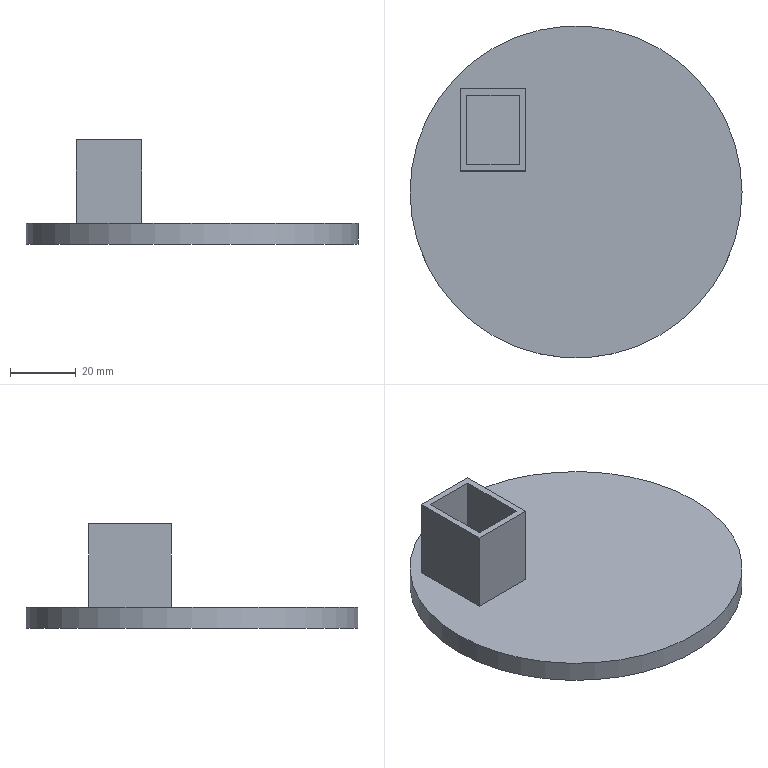Component | NX | BASE | 1 solid | 13 faces | box 101 x 101 x 31.75 mm | volume 55041 mm3 | plane 12 | cylinder 1 | commonest cylinder face diameters 101 x1
STEP:
#1=CARTESIAN_POINT('',(0.,0.,0.));
#2=DIRECTION('',(0.,0.,1.));
#3=DIRECTION('',(1.,0.,0.));
#4=AXIS2_PLACEMENT_3D('',#1,#2,#3);
#5=CARTESIAN_POINT('',(2.788,-28.523,-7.207));
#6=VERTEX_POINT('',#5);
#7=CARTESIAN_POINT('',(22.788,-28.523,-7.207));
#8=VERTEX_POINT('',#7);
#9=CARTESIAN_POINT('',(2.788,-28.523,-7.207));
#10=DIRECTION('',(1.,0.,0.));
#11=VECTOR('',#10,1.);
#12=LINE('',#9,#11);
#13=CARTESIAN_POINT('',(38.028,-34.873,-7.207));
#14=DIRECTION('',(0.,0.,1.));
#15=DIRECTION('',(1.,0.,0.));
#16=AXIS2_PLACEMENT_3D('',#13,#14,#15);
#17=PLANE('',#16);
#18=CARTESIAN_POINT('',(-35.24,6.35));
#19=DIRECTION('',(1.,0.));
#20=VECTOR('',#19,1.);
#21=LINE('',#18,#20);
#22=(GEOMETRIC_REPRESENTATION_CONTEXT(2)PARAMETRIC_REPRESENTATION_CONTEXT()REPRESENTATION_CONTEXT('',''));
#23=DEFINITIONAL_REPRESENTATION('',(#21),#22);
#24=PCURVE('',#17,#23);
#25=CARTESIAN_POINT('',(2.788,-28.523,-7.207));
#26=DIRECTION('',(0.,-1.,0.));
#27=DIRECTION('',(1.,0.,0.));
#28=AXIS2_PLACEMENT_3D('',#25,#26,#27);
#29=PLANE('',#28);
#30=CARTESIAN_POINT('',(0.,0.));
#31=DIRECTION('',(1.,0.));
#32=VECTOR('',#31,1.);
#33=LINE('',#30,#32);
#34=(GEOMETRIC_REPRESENTATION_CONTEXT(2)PARAMETRIC_REPRESENTATION_CONTEXT()REPRESENTATION_CONTEXT('',''));
#35=DEFINITIONAL_REPRESENTATION('',(#33),#34);
#36=PCURVE('',#29,#35);
#37=SURFACE_CURVE('',#12,(#24,#36),.PCURVE_S1.);
#38=EDGE_CURVE('',#6,#8,#37,.T.);
#39=ORIENTED_EDGE('',*,*,#38,.F.);
#40=CARTESIAN_POINT('',(2.788,-3.523,-7.207));
#41=VERTEX_POINT('',#40);
#42=CARTESIAN_POINT('',(2.788,-3.523,-7.207));
#43=DIRECTION('',(0.,-1.,0.));
#44=VECTOR('',#43,1.);
#45=LINE('',#42,#44);
#46=CARTESIAN_POINT('',(-35.24,31.35));
#47=DIRECTION('',(0.,-1.));
#48=VECTOR('',#47,1.);
#49=LINE('',#46,#48);
#50=(GEOMETRIC_REPRESENTATION_CONTEXT(2)PARAMETRIC_REPRESENTATION_CONTEXT()REPRESENTATION_CONTEXT('',''));
#51=DEFINITIONAL_REPRESENTATION('',(#49),#50);
#52=PCURVE('',#17,#51);
#53=CARTESIAN_POINT('',(2.788,-3.523,-7.207));
#54=DIRECTION('',(-1.,-0.,0.));
#55=DIRECTION('',(0.,-1.,0.));
#56=AXIS2_PLACEMENT_3D('',#53,#54,#55);
#57=PLANE('',#56);
#58=CARTESIAN_POINT('',(0.,0.));
#59=DIRECTION('',(1.,0.));
#60=VECTOR('',#59,1.);
#61=LINE('',#58,#60);
#62=(GEOMETRIC_REPRESENTATION_CONTEXT(2)PARAMETRIC_REPRESENTATION_CONTEXT()REPRESENTATION_CONTEXT('',''));
#63=DEFINITIONAL_REPRESENTATION('',(#61),#62);
#64=PCURVE('',#57,#63);
#65=SURFACE_CURVE('',#45,(#52,#64),.PCURVE_S1.);
#66=EDGE_CURVE('',#41,#6,#65,.T.);
#67=ORIENTED_EDGE('',*,*,#66,.F.);
#68=CARTESIAN_POINT('',(22.788,-3.523,-7.207));
#69=VERTEX_POINT('',#68);
#70=CARTESIAN_POINT('',(22.788,-3.523,-7.207));
#71=DIRECTION('',(-1.,0.,0.));
#72=VECTOR('',#71,1.);
#73=LINE('',#70,#72);
#74=CARTESIAN_POINT('',(-15.24,31.35));
#75=DIRECTION('',(-1.,0.));
#76=VECTOR('',#75,1.);
#77=LINE('',#74,#76);
#78=(GEOMETRIC_REPRESENTATION_CONTEXT(2)PARAMETRIC_REPRESENTATION_CONTEXT()REPRESENTATION_CONTEXT('',''));
#79=DEFINITIONAL_REPRESENTATION('',(#77),#78);
#80=PCURVE('',#17,#79);
#81=CARTESIAN_POINT('',(22.788,-3.523,-7.207));
#82=DIRECTION('',(0.,1.,0.));
#83=DIRECTION('',(0.,0.,1.));
#84=AXIS2_PLACEMENT_3D('',#81,#82,#83);
#85=PLANE('',#84);
#86=CARTESIAN_POINT('',(0.,0.));
#87=DIRECTION('',(0.,-1.));
#88=VECTOR('',#87,1.);
#89=LINE('',#86,#88);
#90=(GEOMETRIC_REPRESENTATION_CONTEXT(2)PARAMETRIC_REPRESENTATION_CONTEXT()REPRESENTATION_CONTEXT('',''));
#91=DEFINITIONAL_REPRESENTATION('',(#89),#90);
#92=PCURVE('',#85,#91);
#93=SURFACE_CURVE('',#73,(#80,#92),.PCURVE_S1.);
#94=EDGE_CURVE('',#69,#41,#93,.T.);
#95=ORIENTED_EDGE('',*,*,#94,.F.);
#96=CARTESIAN_POINT('',(22.788,-28.523,-7.207));
#97=DIRECTION('',(-0.,1.,0.));
#98=VECTOR('',#97,1.);
#99=LINE('',#96,#98);
#100=CARTESIAN_POINT('',(-15.24,6.35));
#101=DIRECTION('',(-0.,1.));
#102=VECTOR('',#101,1.);
#103=LINE('',#100,#102);
#104=(GEOMETRIC_REPRESENTATION_CONTEXT(2)PARAMETRIC_REPRESENTATION_CONTEXT()REPRESENTATION_CONTEXT('',''));
#105=DEFINITIONAL_REPRESENTATION('',(#103),#104);
#106=PCURVE('',#17,#105);
#107=CARTESIAN_POINT('',(22.788,-28.523,-7.207));
#108=DIRECTION('',(1.,0.,0.));
#109=DIRECTION('',(-0.,1.,0.));
#110=AXIS2_PLACEMENT_3D('',#107,#108,#109);
#111=PLANE('',#110);
#112=CARTESIAN_POINT('',(0.,0.));
#113=DIRECTION('',(1.,0.));
#114=VECTOR('',#113,1.);
#115=LINE('',#112,#114);
#116=(GEOMETRIC_REPRESENTATION_CONTEXT(2)PARAMETRIC_REPRESENTATION_CONTEXT()REPRESENTATION_CONTEXT('',''));
#117=DEFINITIONAL_REPRESENTATION('',(#115),#116);
#118=PCURVE('',#111,#117);
#119=SURFACE_CURVE('',#99,(#106,#118),.PCURVE_S1.);
#120=EDGE_CURVE('',#8,#69,#119,.T.);
#121=ORIENTED_EDGE('',*,*,#120,.F.);
#122=EDGE_LOOP('',(#39,#67,#95,#121));
#123=FACE_BOUND('',#122,.T.);
#124=CARTESIAN_POINT('',(88.528,-34.873,-7.207));
#125=VERTEX_POINT('',#124);
#126=CARTESIAN_POINT('',(38.028,-34.873,-7.207));
#127=DIRECTION('',(0.,0.,-1.));
#128=DIRECTION('',(1.,0.,0.));
#129=AXIS2_PLACEMENT_3D('',#126,#127,#128);
#130=CIRCLE('',#129,50.5);
#131=CARTESIAN_POINT('',(50.5,0.));
#132=CARTESIAN_POINT('',(50.5,-87.469));
#133=CARTESIAN_POINT('',(-25.25,-43.734));
#134=CARTESIAN_POINT('',(-101.,-0.));
#135=CARTESIAN_POINT('',(-25.25,43.734));
#136=CARTESIAN_POINT('',(50.5,87.469));
#137=CARTESIAN_POINT('',(50.5,0.));
#138=(BOUNDED_CURVE()B_SPLINE_CURVE(2,(#131,#132,#133,#134,#135,#136,#137),.UNSPECIFIED.,.T.,.F.)B_SPLINE_CURVE_WITH_KNOTS((1,2,2,2,2,1),(-2.094,0.,2.094,4.189,6.283,8.378),.UNSPECIFIED.)CURVE()GEOMETRIC_REPRESENTATION_ITEM()RATIONAL_B_SPLINE_CURVE((1.,0.5,1.,0.5,1.,0.5,1.))REPRESENTATION_ITEM(''));
#139=(GEOMETRIC_REPRESENTATION_CONTEXT(2)PARAMETRIC_REPRESENTATION_CONTEXT()REPRESENTATION_CONTEXT('',''));
#140=DEFINITIONAL_REPRESENTATION('',(#138),#139);
#141=PCURVE('',#17,#140);
#142=CARTESIAN_POINT('',(38.028,-34.873,-13.557));
#143=DIRECTION('',(0.,0.,1.));
#144=DIRECTION('',(1.,0.,0.));
#145=AXIS2_PLACEMENT_3D('',#142,#143,#144);
#146=CYLINDRICAL_SURFACE('',#145,50.5);
#147=CARTESIAN_POINT('',(6.283,6.35));
#148=DIRECTION('',(-1.,0.));
#149=VECTOR('',#148,1.);
#150=LINE('',#147,#149);
#151=(GEOMETRIC_REPRESENTATION_CONTEXT(2)PARAMETRIC_REPRESENTATION_CONTEXT()REPRESENTATION_CONTEXT('',''));
#152=DEFINITIONAL_REPRESENTATION('',(#150),#151);
#153=PCURVE('',#146,#152);
#154=SURFACE_CURVE('',#130,(#141,#153),.PCURVE_S1.);
#155=EDGE_CURVE('',#125,#125,#154,.T.);
#156=ORIENTED_EDGE('',*,*,#155,.F.);
#157=EDGE_LOOP('',(#156));
#158=FACE_BOUND('',#157,.T.);
#159=ADVANCED_FACE('',(#123,#158),#17,.T.);
#160=CARTESIAN_POINT('',(88.528,-34.873,-13.557));
#161=VERTEX_POINT('',#160);
#162=CARTESIAN_POINT('',(38.028,-34.873,-13.557));
#163=DIRECTION('',(0.,0.,1.));
#164=DIRECTION('',(1.,0.,0.));
#165=AXIS2_PLACEMENT_3D('',#162,#163,#164);
#166=CIRCLE('',#165,50.5);
#167=CARTESIAN_POINT('',(38.028,-34.873,-13.557));
#168=DIRECTION('',(0.,0.,-1.));
#169=DIRECTION('',(-1.,0.,0.));
#170=AXIS2_PLACEMENT_3D('',#167,#168,#169);
#171=PLANE('',#170);
#172=CARTESIAN_POINT('',(-50.5,0.));
#173=CARTESIAN_POINT('',(-50.5,87.469));
#174=CARTESIAN_POINT('',(25.25,43.734));
#175=CARTESIAN_POINT('',(101.,0.));
#176=CARTESIAN_POINT('',(25.25,-43.734));
#177=CARTESIAN_POINT('',(-50.5,-87.469));
#178=CARTESIAN_POINT('',(-50.5,0.));
#179=(BOUNDED_CURVE()B_SPLINE_CURVE(2,(#172,#173,#174,#175,#176,#177,#178),.UNSPECIFIED.,.T.,.F.)B_SPLINE_CURVE_WITH_KNOTS((1,2,2,2,2,1),(-2.094,0.,2.094,4.189,6.283,8.378),.UNSPECIFIED.)CURVE()GEOMETRIC_REPRESENTATION_ITEM()RATIONAL_B_SPLINE_CURVE((1.,0.5,1.,0.5,1.,0.5,1.))REPRESENTATION_ITEM(''));
#180=(GEOMETRIC_REPRESENTATION_CONTEXT(2)PARAMETRIC_REPRESENTATION_CONTEXT()REPRESENTATION_CONTEXT('',''));
#181=DEFINITIONAL_REPRESENTATION('',(#179),#180);
#182=PCURVE('',#171,#181);
#183=CARTESIAN_POINT('',(0.,0.));
#184=DIRECTION('',(1.,0.));
#185=VECTOR('',#184,1.);
#186=LINE('',#183,#185);
#187=(GEOMETRIC_REPRESENTATION_CONTEXT(2)PARAMETRIC_REPRESENTATION_CONTEXT()REPRESENTATION_CONTEXT('',''));
#188=DEFINITIONAL_REPRESENTATION('',(#186),#187);
#189=PCURVE('',#146,#188);
#190=SURFACE_CURVE('',#166,(#182,#189),.PCURVE_S1.);
#191=EDGE_CURVE('',#161,#161,#190,.T.);
#192=ORIENTED_EDGE('',*,*,#191,.F.);
#193=EDGE_LOOP('',(#192));
#194=FACE_BOUND('',#193,.T.);
#195=ADVANCED_FACE('',(#194),#171,.T.);
#196=ORIENTED_EDGE('',*,*,#155,.T.);
#197=CARTESIAN_POINT('',(88.528,-34.873,-13.557));
#198=CARTESIAN_POINT('',(88.528,-34.873,-7.207));
#199=B_SPLINE_CURVE_WITH_KNOTS('',1,(#197,#198),.UNSPECIFIED.,.F.,.F.,(2,2),(0.,6.35),.PIECEWISE_BEZIER_KNOTS.);
#200=CARTESIAN_POINT('',(0.,0.));
#201=DIRECTION('',(0.,1.));
#202=VECTOR('',#201,1.);
#203=LINE('',#200,#202);
#204=(GEOMETRIC_REPRESENTATION_CONTEXT(2)PARAMETRIC_REPRESENTATION_CONTEXT()REPRESENTATION_CONTEXT('',''));
#205=DEFINITIONAL_REPRESENTATION('',(#203),#204);
#206=PCURVE('',#146,#205);
#207=CARTESIAN_POINT('',(6.283,0.));
#208=DIRECTION('',(0.,1.));
#209=VECTOR('',#208,1.);
#210=LINE('',#207,#209);
#211=(GEOMETRIC_REPRESENTATION_CONTEXT(2)PARAMETRIC_REPRESENTATION_CONTEXT()REPRESENTATION_CONTEXT('',''));
#212=DEFINITIONAL_REPRESENTATION('',(#210),#211);
#213=PCURVE('',#146,#212);
#214=SEAM_CURVE('',#199,(#206,#213),.PCURVE_S1.);
#215=EDGE_CURVE('',#161,#125,#214,.T.);
#216=ORIENTED_EDGE('',*,*,#215,.F.);
#217=ORIENTED_EDGE('',*,*,#191,.T.);
#218=ORIENTED_EDGE('',*,*,#215,.T.);
#219=EDGE_LOOP('',(#196,#216,#217,#218));
#220=FACE_BOUND('',#219,.T.);
#221=ADVANCED_FACE('',(#220),#146,.T.);
#222=CARTESIAN_POINT('',(4.788,-5.523,18.193));
#223=VERTEX_POINT('',#222);
#224=CARTESIAN_POINT('',(4.788,-26.523,18.193));
#225=VERTEX_POINT('',#224);
#226=CARTESIAN_POINT('',(4.788,-3.523,18.193));
#227=DIRECTION('',(0.,-1.,0.));
#228=VECTOR('',#227,1.);
#229=LINE('',#226,#228);
#230=CARTESIAN_POINT('',(22.788,-3.523,18.193));
#231=DIRECTION('',(0.,0.,-1.));
#232=DIRECTION('',(-1.,0.,0.));
#233=AXIS2_PLACEMENT_3D('',#230,#231,#232);
#234=PLANE('',#233);
#235=CARTESIAN_POINT('',(18.,0.));
#236=DIRECTION('',(-0.,-1.));
#237=VECTOR('',#236,1.);
#238=LINE('',#235,#237);
#239=(GEOMETRIC_REPRESENTATION_CONTEXT(2)PARAMETRIC_REPRESENTATION_CONTEXT()REPRESENTATION_CONTEXT('',''));
#240=DEFINITIONAL_REPRESENTATION('',(#238),#239);
#241=PCURVE('',#234,#240);
#242=CARTESIAN_POINT('',(4.788,-3.523,-7.207));
#243=DIRECTION('',(-1.,-0.,0.));
#244=DIRECTION('',(0.,-1.,0.));
#245=AXIS2_PLACEMENT_3D('',#242,#243,#244);
#246=PLANE('',#245);
#247=CARTESIAN_POINT('',(0.,25.4));
#248=DIRECTION('',(1.,0.));
#249=VECTOR('',#248,1.);
#250=LINE('',#247,#249);
#251=(GEOMETRIC_REPRESENTATION_CONTEXT(2)PARAMETRIC_REPRESENTATION_CONTEXT()REPRESENTATION_CONTEXT('',''));
#252=DEFINITIONAL_REPRESENTATION('',(#250),#251);
#253=PCURVE('',#246,#252);
#254=SURFACE_CURVE('',#229,(#241,#253),.PCURVE_S1.);
#255=EDGE_CURVE('',#223,#225,#254,.T.);
#256=ORIENTED_EDGE('',*,*,#255,.F.);
#257=CARTESIAN_POINT('',(20.788,-5.523,18.193));
#258=VERTEX_POINT('',#257);
#259=CARTESIAN_POINT('',(22.788,-5.523,18.193));
#260=DIRECTION('',(-1.,0.,0.));
#261=VECTOR('',#260,1.);
#262=LINE('',#259,#261);
#263=CARTESIAN_POINT('',(0.,-2.));
#264=DIRECTION('',(1.,0.));
#265=VECTOR('',#264,1.);
#266=LINE('',#263,#265);
#267=(GEOMETRIC_REPRESENTATION_CONTEXT(2)PARAMETRIC_REPRESENTATION_CONTEXT()REPRESENTATION_CONTEXT('',''));
#268=DEFINITIONAL_REPRESENTATION('',(#266),#267);
#269=PCURVE('',#234,#268);
#270=CARTESIAN_POINT('',(22.788,-5.523,-7.207));
#271=DIRECTION('',(0.,1.,0.));
#272=DIRECTION('',(0.,0.,1.));
#273=AXIS2_PLACEMENT_3D('',#270,#271,#272);
#274=PLANE('',#273);
#275=CARTESIAN_POINT('',(25.4,0.));
#276=DIRECTION('',(0.,-1.));
#277=VECTOR('',#276,1.);
#278=LINE('',#275,#277);
#279=(GEOMETRIC_REPRESENTATION_CONTEXT(2)PARAMETRIC_REPRESENTATION_CONTEXT()REPRESENTATION_CONTEXT('',''));
#280=DEFINITIONAL_REPRESENTATION('',(#278),#279);
#281=PCURVE('',#274,#280);
#282=SURFACE_CURVE('',#262,(#269,#281),.PCURVE_S1.);
#283=EDGE_CURVE('',#258,#223,#282,.T.);
#284=ORIENTED_EDGE('',*,*,#283,.F.);
#285=CARTESIAN_POINT('',(20.788,-26.523,18.193));
#286=VERTEX_POINT('',#285);
#287=CARTESIAN_POINT('',(20.788,-28.523,18.193));
#288=DIRECTION('',(-0.,1.,0.));
#289=VECTOR('',#288,1.);
#290=LINE('',#287,#289);
#291=CARTESIAN_POINT('',(2.,-25.));
#292=DIRECTION('',(0.,1.));
#293=VECTOR('',#292,1.);
#294=LINE('',#291,#293);
#295=(GEOMETRIC_REPRESENTATION_CONTEXT(2)PARAMETRIC_REPRESENTATION_CONTEXT()REPRESENTATION_CONTEXT('',''));
#296=DEFINITIONAL_REPRESENTATION('',(#294),#295);
#297=PCURVE('',#234,#296);
#298=CARTESIAN_POINT('',(20.788,-28.523,-7.207));
#299=DIRECTION('',(1.,0.,0.));
#300=DIRECTION('',(-0.,1.,0.));
#301=AXIS2_PLACEMENT_3D('',#298,#299,#300);
#302=PLANE('',#301);
#303=CARTESIAN_POINT('',(0.,25.4));
#304=DIRECTION('',(1.,0.));
#305=VECTOR('',#304,1.);
#306=LINE('',#303,#305);
#307=(GEOMETRIC_REPRESENTATION_CONTEXT(2)PARAMETRIC_REPRESENTATION_CONTEXT()REPRESENTATION_CONTEXT('',''));
#308=DEFINITIONAL_REPRESENTATION('',(#306),#307);
#309=PCURVE('',#302,#308);
#310=SURFACE_CURVE('',#290,(#297,#309),.PCURVE_S1.);
#311=EDGE_CURVE('',#286,#258,#310,.T.);
#312=ORIENTED_EDGE('',*,*,#311,.F.);
#313=CARTESIAN_POINT('',(2.788,-26.523,18.193));
#314=DIRECTION('',(1.,0.,0.));
#315=VECTOR('',#314,1.);
#316=LINE('',#313,#315);
#317=CARTESIAN_POINT('',(20.,-23.));
#318=DIRECTION('',(-1.,0.));
#319=VECTOR('',#318,1.);
#320=LINE('',#317,#319);
#321=(GEOMETRIC_REPRESENTATION_CONTEXT(2)PARAMETRIC_REPRESENTATION_CONTEXT()REPRESENTATION_CONTEXT('',''));
#322=DEFINITIONAL_REPRESENTATION('',(#320),#321);
#323=PCURVE('',#234,#322);
#324=CARTESIAN_POINT('',(2.788,-26.523,-7.207));
#325=DIRECTION('',(0.,-1.,0.));
#326=DIRECTION('',(1.,0.,0.));
#327=AXIS2_PLACEMENT_3D('',#324,#325,#326);
#328=PLANE('',#327);
#329=CARTESIAN_POINT('',(0.,25.4));
#330=DIRECTION('',(1.,0.));
#331=VECTOR('',#330,1.);
#332=LINE('',#329,#331);
#333=(GEOMETRIC_REPRESENTATION_CONTEXT(2)PARAMETRIC_REPRESENTATION_CONTEXT()REPRESENTATION_CONTEXT('',''));
#334=DEFINITIONAL_REPRESENTATION('',(#332),#333);
#335=PCURVE('',#328,#334);
#336=SURFACE_CURVE('',#316,(#323,#335),.PCURVE_S1.);
#337=EDGE_CURVE('',#225,#286,#336,.T.);
#338=ORIENTED_EDGE('',*,*,#337,.F.);
#339=EDGE_LOOP('',(#256,#284,#312,#338));
#340=FACE_BOUND('',#339,.T.);
#341=CARTESIAN_POINT('',(22.788,-3.523,18.193));
#342=VERTEX_POINT('',#341);
#343=CARTESIAN_POINT('',(2.788,-3.523,18.193));
#344=VERTEX_POINT('',#343);
#345=CARTESIAN_POINT('',(22.788,-3.523,18.193));
#346=DIRECTION('',(-1.,0.,0.));
#347=VECTOR('',#346,1.);
#348=LINE('',#345,#347);
#349=CARTESIAN_POINT('',(0.,0.));
#350=DIRECTION('',(1.,0.));
#351=VECTOR('',#350,1.);
#352=LINE('',#349,#351);
#353=(GEOMETRIC_REPRESENTATION_CONTEXT(2)PARAMETRIC_REPRESENTATION_CONTEXT()REPRESENTATION_CONTEXT('',''));
#354=DEFINITIONAL_REPRESENTATION('',(#352),#353);
#355=PCURVE('',#234,#354);
#356=CARTESIAN_POINT('',(25.4,0.));
#357=DIRECTION('',(0.,-1.));
#358=VECTOR('',#357,1.);
#359=LINE('',#356,#358);
#360=(GEOMETRIC_REPRESENTATION_CONTEXT(2)PARAMETRIC_REPRESENTATION_CONTEXT()REPRESENTATION_CONTEXT('',''));
#361=DEFINITIONAL_REPRESENTATION('',(#359),#360);
#362=PCURVE('',#85,#361);
#363=SURFACE_CURVE('',#348,(#355,#362),.PCURVE_S1.);
#364=EDGE_CURVE('',#342,#344,#363,.T.);
#365=ORIENTED_EDGE('',*,*,#364,.T.);
#366=CARTESIAN_POINT('',(2.788,-28.523,18.193));
#367=VERTEX_POINT('',#366);
#368=CARTESIAN_POINT('',(2.788,-3.523,18.193));
#369=DIRECTION('',(0.,-1.,0.));
#370=VECTOR('',#369,1.);
#371=LINE('',#368,#370);
#372=CARTESIAN_POINT('',(20.,0.));
#373=DIRECTION('',(-0.,-1.));
#374=VECTOR('',#373,1.);
#375=LINE('',#372,#374);
#376=(GEOMETRIC_REPRESENTATION_CONTEXT(2)PARAMETRIC_REPRESENTATION_CONTEXT()REPRESENTATION_CONTEXT('',''));
#377=DEFINITIONAL_REPRESENTATION('',(#375),#376);
#378=PCURVE('',#234,#377);
#379=CARTESIAN_POINT('',(0.,25.4));
#380=DIRECTION('',(1.,0.));
#381=VECTOR('',#380,1.);
#382=LINE('',#379,#381);
#383=(GEOMETRIC_REPRESENTATION_CONTEXT(2)PARAMETRIC_REPRESENTATION_CONTEXT()REPRESENTATION_CONTEXT('',''));
#384=DEFINITIONAL_REPRESENTATION('',(#382),#383);
#385=PCURVE('',#57,#384);
#386=SURFACE_CURVE('',#371,(#378,#385),.PCURVE_S1.);
#387=EDGE_CURVE('',#344,#367,#386,.T.);
#388=ORIENTED_EDGE('',*,*,#387,.T.);
#389=CARTESIAN_POINT('',(22.788,-28.523,18.193));
#390=VERTEX_POINT('',#389);
#391=CARTESIAN_POINT('',(2.788,-28.523,18.193));
#392=DIRECTION('',(1.,0.,0.));
#393=VECTOR('',#392,1.);
#394=LINE('',#391,#393);
#395=CARTESIAN_POINT('',(20.,-25.));
#396=DIRECTION('',(-1.,0.));
#397=VECTOR('',#396,1.);
#398=LINE('',#395,#397);
#399=(GEOMETRIC_REPRESENTATION_CONTEXT(2)PARAMETRIC_REPRESENTATION_CONTEXT()REPRESENTATION_CONTEXT('',''));
#400=DEFINITIONAL_REPRESENTATION('',(#398),#399);
#401=PCURVE('',#234,#400);
#402=CARTESIAN_POINT('',(0.,25.4));
#403=DIRECTION('',(1.,0.));
#404=VECTOR('',#403,1.);
#405=LINE('',#402,#404);
#406=(GEOMETRIC_REPRESENTATION_CONTEXT(2)PARAMETRIC_REPRESENTATION_CONTEXT()REPRESENTATION_CONTEXT('',''));
#407=DEFINITIONAL_REPRESENTATION('',(#405),#406);
#408=PCURVE('',#29,#407);
#409=SURFACE_CURVE('',#394,(#401,#408),.PCURVE_S1.);
#410=EDGE_CURVE('',#367,#390,#409,.T.);
#411=ORIENTED_EDGE('',*,*,#410,.T.);
#412=CARTESIAN_POINT('',(22.788,-28.523,18.193));
#413=DIRECTION('',(-0.,1.,0.));
#414=VECTOR('',#413,1.);
#415=LINE('',#412,#414);
#416=CARTESIAN_POINT('',(-0.,-25.));
#417=DIRECTION('',(0.,1.));
#418=VECTOR('',#417,1.);
#419=LINE('',#416,#418);
#420=(GEOMETRIC_REPRESENTATION_CONTEXT(2)PARAMETRIC_REPRESENTATION_CONTEXT()REPRESENTATION_CONTEXT('',''));
#421=DEFINITIONAL_REPRESENTATION('',(#419),#420);
#422=PCURVE('',#234,#421);
#423=CARTESIAN_POINT('',(0.,25.4));
#424=DIRECTION('',(1.,0.));
#425=VECTOR('',#424,1.);
#426=LINE('',#423,#425);
#427=(GEOMETRIC_REPRESENTATION_CONTEXT(2)PARAMETRIC_REPRESENTATION_CONTEXT()REPRESENTATION_CONTEXT('',''));
#428=DEFINITIONAL_REPRESENTATION('',(#426),#427);
#429=PCURVE('',#111,#428);
#430=SURFACE_CURVE('',#415,(#422,#429),.PCURVE_S1.);
#431=EDGE_CURVE('',#390,#342,#430,.T.);
#432=ORIENTED_EDGE('',*,*,#431,.T.);
#433=EDGE_LOOP('',(#365,#388,#411,#432));
#434=FACE_BOUND('',#433,.T.);
#435=ADVANCED_FACE('',(#340,#434),#234,.F.);
#436=ORIENTED_EDGE('',*,*,#255,.T.);
#437=CARTESIAN_POINT('',(4.788,-26.523,-7.207));
#438=VERTEX_POINT('',#437);
#439=CARTESIAN_POINT('',(4.788,-26.523,-7.207));
#440=DIRECTION('',(0.,0.,1.));
#441=VECTOR('',#440,1.);
#442=LINE('',#439,#441);
#443=CARTESIAN_POINT('',(23.,0.));
#444=DIRECTION('',(0.,1.));
#445=VECTOR('',#444,1.);
#446=LINE('',#443,#445);
#447=(GEOMETRIC_REPRESENTATION_CONTEXT(2)PARAMETRIC_REPRESENTATION_CONTEXT()REPRESENTATION_CONTEXT('',''));
#448=DEFINITIONAL_REPRESENTATION('',(#446),#447);
#449=PCURVE('',#246,#448);
#450=CARTESIAN_POINT('',(2.,0.));
#451=DIRECTION('',(0.,1.));
#452=VECTOR('',#451,1.);
#453=LINE('',#450,#452);
#454=(GEOMETRIC_REPRESENTATION_CONTEXT(2)PARAMETRIC_REPRESENTATION_CONTEXT()REPRESENTATION_CONTEXT('',''));
#455=DEFINITIONAL_REPRESENTATION('',(#453),#454);
#456=PCURVE('',#328,#455);
#457=SURFACE_CURVE('',#442,(#449,#456),.PCURVE_S1.);
#458=EDGE_CURVE('',#438,#225,#457,.T.);
#459=ORIENTED_EDGE('',*,*,#458,.F.);
#460=CARTESIAN_POINT('',(4.788,-5.523,-7.207));
#461=VERTEX_POINT('',#460);
#462=CARTESIAN_POINT('',(4.788,-3.523,-7.207));
#463=DIRECTION('',(0.,-1.,0.));
#464=VECTOR('',#463,1.);
#465=LINE('',#462,#464);
#466=CARTESIAN_POINT('',(0.,0.));
#467=DIRECTION('',(1.,0.));
#468=VECTOR('',#467,1.);
#469=LINE('',#466,#468);
#470=(GEOMETRIC_REPRESENTATION_CONTEXT(2)PARAMETRIC_REPRESENTATION_CONTEXT()REPRESENTATION_CONTEXT('',''));
#471=DEFINITIONAL_REPRESENTATION('',(#469),#470);
#472=PCURVE('',#246,#471);
#473=CARTESIAN_POINT('',(38.028,-34.873,-7.207));
#474=DIRECTION('',(0.,0.,1.));
#475=DIRECTION('',(1.,0.,0.));
#476=AXIS2_PLACEMENT_3D('',#473,#474,#475);
#477=PLANE('',#476);
#478=CARTESIAN_POINT('',(-33.24,31.35));
#479=DIRECTION('',(0.,-1.));
#480=VECTOR('',#479,1.);
#481=LINE('',#478,#480);
#482=(GEOMETRIC_REPRESENTATION_CONTEXT(2)PARAMETRIC_REPRESENTATION_CONTEXT()REPRESENTATION_CONTEXT('',''));
#483=DEFINITIONAL_REPRESENTATION('',(#481),#482);
#484=PCURVE('',#477,#483);
#485=SURFACE_CURVE('',#465,(#472,#484),.PCURVE_S1.);
#486=EDGE_CURVE('',#461,#438,#485,.T.);
#487=ORIENTED_EDGE('',*,*,#486,.F.);
#488=CARTESIAN_POINT('',(4.788,-5.523,-7.207));
#489=DIRECTION('',(0.,0.,1.));
#490=VECTOR('',#489,1.);
#491=LINE('',#488,#490);
#492=CARTESIAN_POINT('',(2.,0.));
#493=DIRECTION('',(0.,1.));
#494=VECTOR('',#493,1.);
#495=LINE('',#492,#494);
#496=(GEOMETRIC_REPRESENTATION_CONTEXT(2)PARAMETRIC_REPRESENTATION_CONTEXT()REPRESENTATION_CONTEXT('',''));
#497=DEFINITIONAL_REPRESENTATION('',(#495),#496);
#498=PCURVE('',#246,#497);
#499=CARTESIAN_POINT('',(0.,-18.));
#500=DIRECTION('',(1.,0.));
#501=VECTOR('',#500,1.);
#502=LINE('',#499,#501);
#503=(GEOMETRIC_REPRESENTATION_CONTEXT(2)PARAMETRIC_REPRESENTATION_CONTEXT()REPRESENTATION_CONTEXT('',''));
#504=DEFINITIONAL_REPRESENTATION('',(#502),#503);
#505=PCURVE('',#274,#504);
#506=SURFACE_CURVE('',#491,(#498,#505),.PCURVE_S1.);
#507=EDGE_CURVE('',#461,#223,#506,.T.);
#508=ORIENTED_EDGE('',*,*,#507,.T.);
#509=EDGE_LOOP('',(#436,#459,#487,#508));
#510=FACE_BOUND('',#509,.T.);
#511=ADVANCED_FACE('',(#510),#246,.F.);
#512=ORIENTED_EDGE('',*,*,#337,.T.);
#513=CARTESIAN_POINT('',(20.788,-26.523,-7.207));
#514=VERTEX_POINT('',#513);
#515=CARTESIAN_POINT('',(20.788,-26.523,-7.207));
#516=DIRECTION('',(0.,0.,1.));
#517=VECTOR('',#516,1.);
#518=LINE('',#515,#517);
#519=CARTESIAN_POINT('',(18.,0.));
#520=DIRECTION('',(0.,1.));
#521=VECTOR('',#520,1.);
#522=LINE('',#519,#521);
#523=(GEOMETRIC_REPRESENTATION_CONTEXT(2)PARAMETRIC_REPRESENTATION_CONTEXT()REPRESENTATION_CONTEXT('',''));
#524=DEFINITIONAL_REPRESENTATION('',(#522),#523);
#525=PCURVE('',#328,#524);
#526=CARTESIAN_POINT('',(2.,0.));
#527=DIRECTION('',(0.,1.));
#528=VECTOR('',#527,1.);
#529=LINE('',#526,#528);
#530=(GEOMETRIC_REPRESENTATION_CONTEXT(2)PARAMETRIC_REPRESENTATION_CONTEXT()REPRESENTATION_CONTEXT('',''));
#531=DEFINITIONAL_REPRESENTATION('',(#529),#530);
#532=PCURVE('',#302,#531);
#533=SURFACE_CURVE('',#518,(#525,#532),.PCURVE_S1.);
#534=EDGE_CURVE('',#514,#286,#533,.T.);
#535=ORIENTED_EDGE('',*,*,#534,.F.);
#536=CARTESIAN_POINT('',(2.788,-26.523,-7.207));
#537=DIRECTION('',(1.,0.,0.));
#538=VECTOR('',#537,1.);
#539=LINE('',#536,#538);
#540=CARTESIAN_POINT('',(0.,0.));
#541=DIRECTION('',(1.,0.));
#542=VECTOR('',#541,1.);
#543=LINE('',#540,#542);
#544=(GEOMETRIC_REPRESENTATION_CONTEXT(2)PARAMETRIC_REPRESENTATION_CONTEXT()REPRESENTATION_CONTEXT('',''));
#545=DEFINITIONAL_REPRESENTATION('',(#543),#544);
#546=PCURVE('',#328,#545);
#547=CARTESIAN_POINT('',(-35.24,8.35));
#548=DIRECTION('',(1.,0.));
#549=VECTOR('',#548,1.);
#550=LINE('',#547,#549);
#551=(GEOMETRIC_REPRESENTATION_CONTEXT(2)PARAMETRIC_REPRESENTATION_CONTEXT()REPRESENTATION_CONTEXT('',''));
#552=DEFINITIONAL_REPRESENTATION('',(#550),#551);
#553=PCURVE('',#477,#552);
#554=SURFACE_CURVE('',#539,(#546,#553),.PCURVE_S1.);
#555=EDGE_CURVE('',#438,#514,#554,.T.);
#556=ORIENTED_EDGE('',*,*,#555,.F.);
#557=ORIENTED_EDGE('',*,*,#458,.T.);
#558=EDGE_LOOP('',(#512,#535,#556,#557));
#559=FACE_BOUND('',#558,.T.);
#560=ADVANCED_FACE('',(#559),#328,.F.);
#561=ORIENTED_EDGE('',*,*,#311,.T.);
#562=CARTESIAN_POINT('',(20.788,-5.523,-7.207));
#563=VERTEX_POINT('',#562);
#564=CARTESIAN_POINT('',(20.788,-5.523,-7.207));
#565=DIRECTION('',(0.,0.,1.));
#566=VECTOR('',#565,1.);
#567=LINE('',#564,#566);
#568=CARTESIAN_POINT('',(23.,0.));
#569=DIRECTION('',(0.,1.));
#570=VECTOR('',#569,1.);
#571=LINE('',#568,#570);
#572=(GEOMETRIC_REPRESENTATION_CONTEXT(2)PARAMETRIC_REPRESENTATION_CONTEXT()REPRESENTATION_CONTEXT('',''));
#573=DEFINITIONAL_REPRESENTATION('',(#571),#572);
#574=PCURVE('',#302,#573);
#575=CARTESIAN_POINT('',(0.,-2.));
#576=DIRECTION('',(1.,0.));
#577=VECTOR('',#576,1.);
#578=LINE('',#575,#577);
#579=(GEOMETRIC_REPRESENTATION_CONTEXT(2)PARAMETRIC_REPRESENTATION_CONTEXT()REPRESENTATION_CONTEXT('',''));
#580=DEFINITIONAL_REPRESENTATION('',(#578),#579);
#581=PCURVE('',#274,#580);
#582=SURFACE_CURVE('',#567,(#574,#581),.PCURVE_S1.);
#583=EDGE_CURVE('',#563,#258,#582,.T.);
#584=ORIENTED_EDGE('',*,*,#583,.F.);
#585=CARTESIAN_POINT('',(20.788,-28.523,-7.207));
#586=DIRECTION('',(-0.,1.,0.));
#587=VECTOR('',#586,1.);
#588=LINE('',#585,#587);
#589=CARTESIAN_POINT('',(0.,0.));
#590=DIRECTION('',(1.,0.));
#591=VECTOR('',#590,1.);
#592=LINE('',#589,#591);
#593=(GEOMETRIC_REPRESENTATION_CONTEXT(2)PARAMETRIC_REPRESENTATION_CONTEXT()REPRESENTATION_CONTEXT('',''));
#594=DEFINITIONAL_REPRESENTATION('',(#592),#593);
#595=PCURVE('',#302,#594);
#596=CARTESIAN_POINT('',(-17.24,6.35));
#597=DIRECTION('',(-0.,1.));
#598=VECTOR('',#597,1.);
#599=LINE('',#596,#598);
#600=(GEOMETRIC_REPRESENTATION_CONTEXT(2)PARAMETRIC_REPRESENTATION_CONTEXT()REPRESENTATION_CONTEXT('',''));
#601=DEFINITIONAL_REPRESENTATION('',(#599),#600);
#602=PCURVE('',#477,#601);
#603=SURFACE_CURVE('',#588,(#595,#602),.PCURVE_S1.);
#604=EDGE_CURVE('',#514,#563,#603,.T.);
#605=ORIENTED_EDGE('',*,*,#604,.F.);
#606=ORIENTED_EDGE('',*,*,#534,.T.);
#607=EDGE_LOOP('',(#561,#584,#605,#606));
#608=FACE_BOUND('',#607,.T.);
#609=ADVANCED_FACE('',(#608),#302,.F.);
#610=ORIENTED_EDGE('',*,*,#283,.T.);
#611=ORIENTED_EDGE('',*,*,#507,.F.);
#612=CARTESIAN_POINT('',(22.788,-5.523,-7.207));
#613=DIRECTION('',(-1.,0.,0.));
#614=VECTOR('',#613,1.);
#615=LINE('',#612,#614);
#616=CARTESIAN_POINT('',(0.,0.));
#617=DIRECTION('',(0.,-1.));
#618=VECTOR('',#617,1.);
#619=LINE('',#616,#618);
#620=(GEOMETRIC_REPRESENTATION_CONTEXT(2)PARAMETRIC_REPRESENTATION_CONTEXT()REPRESENTATION_CONTEXT('',''));
#621=DEFINITIONAL_REPRESENTATION('',(#619),#620);
#622=PCURVE('',#274,#621);
#623=CARTESIAN_POINT('',(-15.24,29.35));
#624=DIRECTION('',(-1.,0.));
#625=VECTOR('',#624,1.);
#626=LINE('',#623,#625);
#627=(GEOMETRIC_REPRESENTATION_CONTEXT(2)PARAMETRIC_REPRESENTATION_CONTEXT()REPRESENTATION_CONTEXT('',''));
#628=DEFINITIONAL_REPRESENTATION('',(#626),#627);
#629=PCURVE('',#477,#628);
#630=SURFACE_CURVE('',#615,(#622,#629),.PCURVE_S1.);
#631=EDGE_CURVE('',#563,#461,#630,.T.);
#632=ORIENTED_EDGE('',*,*,#631,.F.);
#633=ORIENTED_EDGE('',*,*,#583,.T.);
#634=EDGE_LOOP('',(#610,#611,#632,#633));
#635=FACE_BOUND('',#634,.T.);
#636=ADVANCED_FACE('',(#635),#274,.F.);
#637=ORIENTED_EDGE('',*,*,#387,.F.);
#638=CARTESIAN_POINT('',(2.788,-3.523,-7.207));
#639=DIRECTION('',(0.,0.,1.));
#640=VECTOR('',#639,1.);
#641=LINE('',#638,#640);
#642=CARTESIAN_POINT('',(0.,0.));
#643=DIRECTION('',(0.,1.));
#644=VECTOR('',#643,1.);
#645=LINE('',#642,#644);
#646=(GEOMETRIC_REPRESENTATION_CONTEXT(2)PARAMETRIC_REPRESENTATION_CONTEXT()REPRESENTATION_CONTEXT('',''));
#647=DEFINITIONAL_REPRESENTATION('',(#645),#646);
#648=PCURVE('',#57,#647);
#649=CARTESIAN_POINT('',(0.,-20.));
#650=DIRECTION('',(1.,0.));
#651=VECTOR('',#650,1.);
#652=LINE('',#649,#651);
#653=(GEOMETRIC_REPRESENTATION_CONTEXT(2)PARAMETRIC_REPRESENTATION_CONTEXT()REPRESENTATION_CONTEXT('',''));
#654=DEFINITIONAL_REPRESENTATION('',(#652),#653);
#655=PCURVE('',#85,#654);
#656=SURFACE_CURVE('',#641,(#648,#655),.PCURVE_S1.);
#657=EDGE_CURVE('',#41,#344,#656,.T.);
#658=ORIENTED_EDGE('',*,*,#657,.F.);
#659=ORIENTED_EDGE('',*,*,#66,.T.);
#660=CARTESIAN_POINT('',(2.788,-28.523,-7.207));
#661=DIRECTION('',(0.,0.,1.));
#662=VECTOR('',#661,1.);
#663=LINE('',#660,#662);
#664=CARTESIAN_POINT('',(25.,0.));
#665=DIRECTION('',(0.,1.));
#666=VECTOR('',#665,1.);
#667=LINE('',#664,#666);
#668=(GEOMETRIC_REPRESENTATION_CONTEXT(2)PARAMETRIC_REPRESENTATION_CONTEXT()REPRESENTATION_CONTEXT('',''));
#669=DEFINITIONAL_REPRESENTATION('',(#667),#668);
#670=PCURVE('',#57,#669);
#671=CARTESIAN_POINT('',(0.,0.));
#672=DIRECTION('',(0.,1.));
#673=VECTOR('',#672,1.);
#674=LINE('',#671,#673);
#675=(GEOMETRIC_REPRESENTATION_CONTEXT(2)PARAMETRIC_REPRESENTATION_CONTEXT()REPRESENTATION_CONTEXT('',''));
#676=DEFINITIONAL_REPRESENTATION('',(#674),#675);
#677=PCURVE('',#29,#676);
#678=SURFACE_CURVE('',#663,(#670,#677),.PCURVE_S1.);
#679=EDGE_CURVE('',#6,#367,#678,.T.);
#680=ORIENTED_EDGE('',*,*,#679,.T.);
#681=EDGE_LOOP('',(#637,#658,#659,#680));
#682=FACE_BOUND('',#681,.T.);
#683=ADVANCED_FACE('',(#682),#57,.T.);
#684=ORIENTED_EDGE('',*,*,#410,.F.);
#685=ORIENTED_EDGE('',*,*,#679,.F.);
#686=ORIENTED_EDGE('',*,*,#38,.T.);
#687=CARTESIAN_POINT('',(22.788,-28.523,-7.207));
#688=DIRECTION('',(0.,0.,1.));
#689=VECTOR('',#688,1.);
#690=LINE('',#687,#689);
#691=CARTESIAN_POINT('',(20.,0.));
#692=DIRECTION('',(0.,1.));
#693=VECTOR('',#692,1.);
#694=LINE('',#691,#693);
#695=(GEOMETRIC_REPRESENTATION_CONTEXT(2)PARAMETRIC_REPRESENTATION_CONTEXT()REPRESENTATION_CONTEXT('',''));
#696=DEFINITIONAL_REPRESENTATION('',(#694),#695);
#697=PCURVE('',#29,#696);
#698=CARTESIAN_POINT('',(0.,0.));
#699=DIRECTION('',(0.,1.));
#700=VECTOR('',#699,1.);
#701=LINE('',#698,#700);
#702=(GEOMETRIC_REPRESENTATION_CONTEXT(2)PARAMETRIC_REPRESENTATION_CONTEXT()REPRESENTATION_CONTEXT('',''));
#703=DEFINITIONAL_REPRESENTATION('',(#701),#702);
#704=PCURVE('',#111,#703);
#705=SURFACE_CURVE('',#690,(#697,#704),.PCURVE_S1.);
#706=EDGE_CURVE('',#8,#390,#705,.T.);
#707=ORIENTED_EDGE('',*,*,#706,.T.);
#708=EDGE_LOOP('',(#684,#685,#686,#707));
#709=FACE_BOUND('',#708,.T.);
#710=ADVANCED_FACE('',(#709),#29,.T.);
#711=ORIENTED_EDGE('',*,*,#431,.F.);
#712=ORIENTED_EDGE('',*,*,#706,.F.);
#713=ORIENTED_EDGE('',*,*,#120,.T.);
#714=CARTESIAN_POINT('',(22.788,-3.523,-7.207));
#715=DIRECTION('',(0.,0.,1.));
#716=VECTOR('',#715,1.);
#717=LINE('',#714,#716);
#718=CARTESIAN_POINT('',(25.,0.));
#719=DIRECTION('',(0.,1.));
#720=VECTOR('',#719,1.);
#721=LINE('',#718,#720);
#722=(GEOMETRIC_REPRESENTATION_CONTEXT(2)PARAMETRIC_REPRESENTATION_CONTEXT()REPRESENTATION_CONTEXT('',''));
#723=DEFINITIONAL_REPRESENTATION('',(#721),#722);
#724=PCURVE('',#111,#723);
#725=CARTESIAN_POINT('',(0.,0.));
#726=DIRECTION('',(1.,0.));
#727=VECTOR('',#726,1.);
#728=LINE('',#725,#727);
#729=(GEOMETRIC_REPRESENTATION_CONTEXT(2)PARAMETRIC_REPRESENTATION_CONTEXT()REPRESENTATION_CONTEXT('',''));
#730=DEFINITIONAL_REPRESENTATION('',(#728),#729);
#731=PCURVE('',#85,#730);
#732=SURFACE_CURVE('',#717,(#724,#731),.PCURVE_S1.);
#733=EDGE_CURVE('',#69,#342,#732,.T.);
#734=ORIENTED_EDGE('',*,*,#733,.T.);
#735=EDGE_LOOP('',(#711,#712,#713,#734));
#736=FACE_BOUND('',#735,.T.);
#737=ADVANCED_FACE('',(#736),#111,.T.);
#738=ORIENTED_EDGE('',*,*,#364,.F.);
#739=ORIENTED_EDGE('',*,*,#733,.F.);
#740=ORIENTED_EDGE('',*,*,#94,.T.);
#741=ORIENTED_EDGE('',*,*,#657,.T.);
#742=EDGE_LOOP('',(#738,#739,#740,#741));
#743=FACE_BOUND('',#742,.T.);
#744=ADVANCED_FACE('',(#743),#85,.T.);
#745=ORIENTED_EDGE('',*,*,#631,.T.);
#746=ORIENTED_EDGE('',*,*,#486,.T.);
#747=ORIENTED_EDGE('',*,*,#555,.T.);
#748=ORIENTED_EDGE('',*,*,#604,.T.);
#749=EDGE_LOOP('',(#745,#746,#747,#748));
#750=FACE_BOUND('',#749,.T.);
#751=ADVANCED_FACE('',(#750),#477,.T.);
#752=CLOSED_SHELL('',(#159,#195,#221,#435,#511,#560,#609,#636,#683,#710,#737,#744,#751));
#753=MANIFOLD_SOLID_BREP('',#752);
#754=(LENGTH_UNIT()NAMED_UNIT(*)SI_UNIT(.MILLI.,.METRE.));
#755=UNCERTAINTY_MEASURE_WITH_UNIT(LENGTH_MEASURE(0.000001),#754,'','');
#756=(NAMED_UNIT(*)PLANE_ANGLE_UNIT()SI_UNIT($,.RADIAN.));
#757=(NAMED_UNIT(*)SI_UNIT($,.STERADIAN.)SOLID_ANGLE_UNIT());
#758=(GEOMETRIC_REPRESENTATION_CONTEXT(3)GLOBAL_UNCERTAINTY_ASSIGNED_CONTEXT((#755))GLOBAL_UNIT_ASSIGNED_CONTEXT((#754,#756,#757))REPRESENTATION_CONTEXT('',''));
#759=ADVANCED_BREP_SHAPE_REPRESENTATION('',(#4,#753),#758);